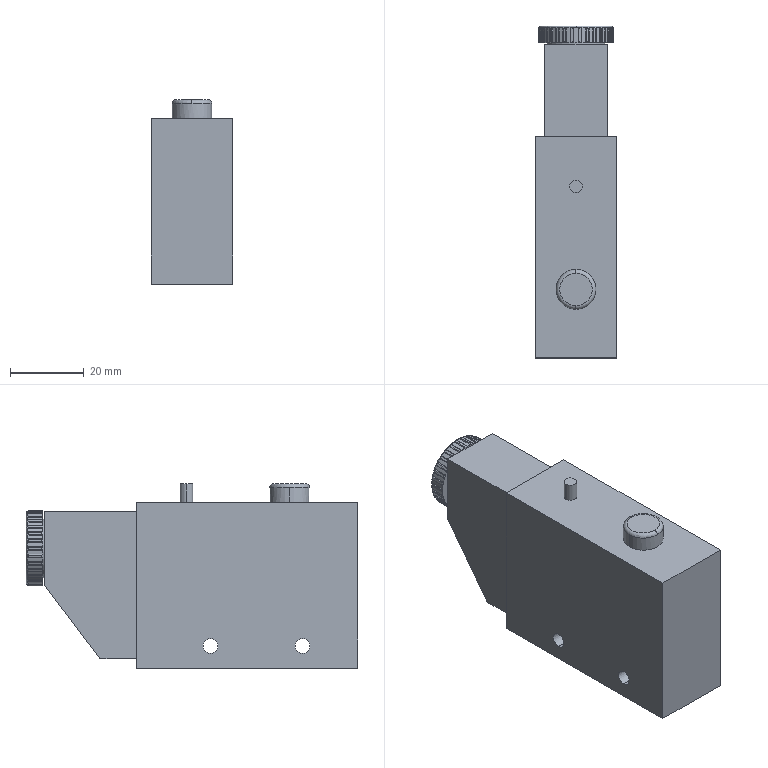Component | SolidWorks | PhotoelectricSensor-1 | 1 solid | 230 faces | volume 75277 mm3 | cylinder 179 | plane 47 | torus 4 | commonest cylinder face diameters 0.4 x136 20 x31 4 x4 10.792 x2 3.449 x2 16 x2 18 x2